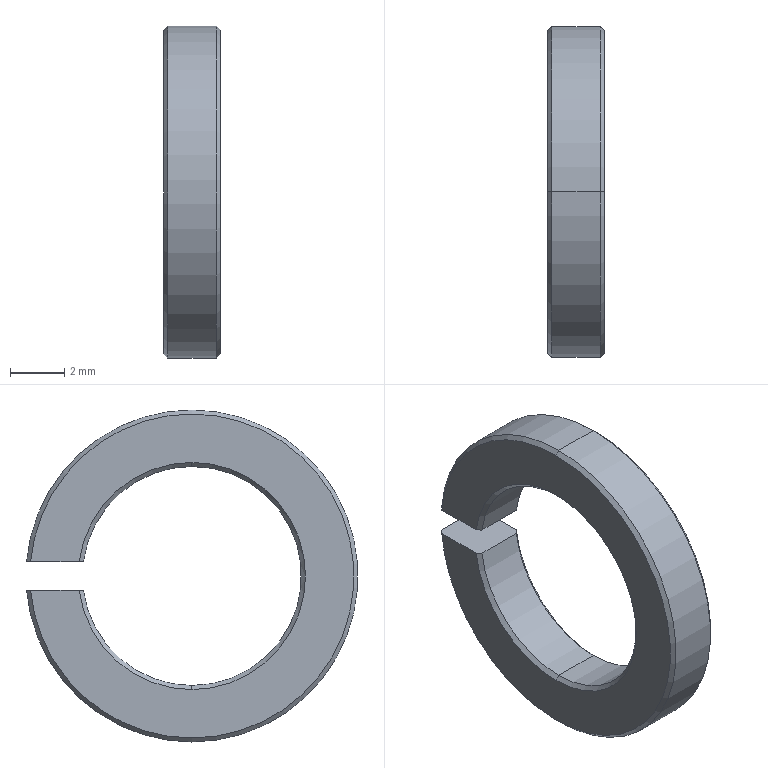Component | SolidWorks | 8_T93-1 | 1 solid | 22 faces | box 2.1 x 12.25 x 12.28 mm | volume 134 mm3 | cone 12 | cylinder 6 | plane 4 | commonest cylinder face diameters 8.1 x3 12.277 x3 | material Plain Carbon Steel
build123d program:
from build123d import *

# Parameters (mm, degrees)
EXTRUDE1_DEPTH = 2.1
CHAMFER1_SIZE  = 0.15


with BuildPart() as part:
    # Sketch1 → Extrude1 (new body)
    with BuildSketch(Plane.XY):
        with BuildLine():
            Line((-0.525, 6.116), (-0.525, 4.016))
            ThreePointArc((-0.525, 4.016), (0, -4.05), (0.525, 4.016))
            Line((0.525, 4.016), (0.525, 6.116))
            ThreePointArc((0.525, 6.116), (0, -6.138), (-0.525, 6.116))
        make_face()
    extrude(amount=EXTRUDE1_DEPTH)

    # Chamfer1
    chamfer1_edges = [part.edges().sort_by_distance(p)[0] for p in [
        (0, -4.05, 2.1),
        (0, -6.138, 2.1),
        (0, -4.05, 0),
        (0, -6.138, 0),
    ]]
    chamfer(chamfer1_edges, length=CHAMFER1_SIZE)


solid = part.part

# Placed as in the assembly
solid = solid.moved(Location((-16.1, 42.426, 42.426), (0, 90, 0)))
STEP:
#1=COLOUR_RGB('',0.7922,0.8196,0.9333);
#2=FILL_AREA_STYLE_COLOUR('',#1);
#3=FILL_AREA_STYLE('',(#2));
#4=SURFACE_STYLE_FILL_AREA(#3);
#5=SURFACE_SIDE_STYLE('',(#4));
#6=SURFACE_STYLE_USAGE(.BOTH.,#5);
#7=PRESENTATION_STYLE_ASSIGNMENT((#6));
#8=CARTESIAN_POINT('',(-0.6339,1.67,1.906));
#9=VERTEX_POINT('',#8);
#10=CARTESIAN_POINT('',(-0.6339,1.905,1.691));
#11=VERTEX_POINT('',#10);
#12=CARTESIAN_POINT('',(-0.6339,1.67,1.67));
#13=DIRECTION('',(-1.,0.,0.));
#14=DIRECTION('',(0.,0.,1.));
#15=AXIS2_PLACEMENT_3D('',#12,#13,#14);
#16=CIRCLE('',#15,0.2358);
#17=EDGE_CURVE('',#9,#11,#16,.T.);
#18=ORIENTED_EDGE('',*,*,#17,.F.);
#19=CARTESIAN_POINT('',(-0.628,1.67,1.912));
#20=VERTEX_POINT('',#19);
#21=CARTESIAN_POINT('',(-0.6339,1.67,1.906));
#22=DIRECTION('',(0.7071,0.,0.7071));
#23=VECTOR('',#22,39.37);
#24=LINE('',#21,#23);
#25=EDGE_CURVE('',#9,#20,#24,.T.);
#26=ORIENTED_EDGE('',*,*,#25,.T.);
#27=CARTESIAN_POINT('',(-0.628,1.911,1.691));
#28=VERTEX_POINT('',#27);
#29=CARTESIAN_POINT('',(-0.628,1.67,1.67));
#30=DIRECTION('',(1.,0.,0.));
#31=DIRECTION('',(0.,0.,1.));
#32=AXIS2_PLACEMENT_3D('',#29,#30,#31);
#33=CIRCLE('',#32,0.2417);
#34=EDGE_CURVE('',#28,#20,#33,.T.);
#35=ORIENTED_EDGE('',*,*,#34,.F.);
#36=CARTESIAN_POINT('',(-0.6339,1.905,1.691));
#37=CARTESIAN_POINT('',(-0.6319,1.907,1.691));
#38=CARTESIAN_POINT('',(-0.6299,1.909,1.691));
#39=CARTESIAN_POINT('',(-0.628,1.911,1.691));
#40=B_SPLINE_CURVE_WITH_KNOTS('',3,(#36,#37,#38,#39),.UNSPECIFIED.,.F.,.F.,(4,4),(0.,0.0002125),.UNSPECIFIED.);
#41=EDGE_CURVE('',#11,#28,#40,.T.);
#42=ORIENTED_EDGE('',*,*,#41,.F.);
#43=EDGE_LOOP('',(#18,#26,#35,#42));
#44=FACE_OUTER_BOUND('',#43,.T.);
#45=CARTESIAN_POINT('',(-0.6339,1.67,1.67));
#46=DIRECTION('',(1.,0.,0.));
#47=DIRECTION('',(0.,0.,-1.));
#48=AXIS2_PLACEMENT_3D('',#45,#46,#47);
#49=CONICAL_SURFACE('',#48,0.2358,0.7854);
#50=ADVANCED_FACE('',(#44),#49,.T.);
#51=ORIENTED_EDGE('',*,*,#25,.F.);
#52=CARTESIAN_POINT('',(-0.6339,1.67,1.435));
#53=VERTEX_POINT('',#52);
#54=CARTESIAN_POINT('',(-0.6339,1.67,1.67));
#55=DIRECTION('',(-1.,0.,0.));
#56=DIRECTION('',(0.,0.,1.));
#57=AXIS2_PLACEMENT_3D('',#54,#55,#56);
#58=CIRCLE('',#57,0.2358);
#59=EDGE_CURVE('',#53,#9,#58,.T.);
#60=ORIENTED_EDGE('',*,*,#59,.F.);
#61=CARTESIAN_POINT('',(-0.628,1.67,1.429));
#62=VERTEX_POINT('',#61);
#63=CARTESIAN_POINT('',(-0.6339,1.67,1.435));
#64=DIRECTION('',(0.7071,0.,-0.7071));
#65=VECTOR('',#64,39.37);
#66=LINE('',#63,#65);
#67=EDGE_CURVE('',#53,#62,#66,.T.);
#68=ORIENTED_EDGE('',*,*,#67,.T.);
#69=CARTESIAN_POINT('',(-0.628,1.67,1.67));
#70=DIRECTION('',(1.,0.,0.));
#71=DIRECTION('',(0.,0.,1.));
#72=AXIS2_PLACEMENT_3D('',#69,#70,#71);
#73=CIRCLE('',#72,0.2417);
#74=EDGE_CURVE('',#20,#62,#73,.T.);
#75=ORIENTED_EDGE('',*,*,#74,.F.);
#76=EDGE_LOOP('',(#51,#60,#68,#75));
#77=FACE_OUTER_BOUND('',#76,.T.);
#78=CARTESIAN_POINT('',(-0.6339,1.67,1.67));
#79=DIRECTION('',(1.,0.,0.));
#80=DIRECTION('',(0.,0.,-1.));
#81=AXIS2_PLACEMENT_3D('',#78,#79,#80);
#82=CONICAL_SURFACE('',#81,0.2358,0.7854);
#83=ADVANCED_FACE('',(#77),#82,.T.);
#84=CARTESIAN_POINT('',(-0.628,1.67,1.511));
#85=VERTEX_POINT('',#84);
#86=CARTESIAN_POINT('',(-0.628,1.67,1.83));
#87=VERTEX_POINT('',#86);
#88=CARTESIAN_POINT('',(-0.628,1.67,1.67));
#89=DIRECTION('',(-1.,0.,0.));
#90=DIRECTION('',(0.,0.,1.));
#91=AXIS2_PLACEMENT_3D('',#88,#89,#90);
#92=CIRCLE('',#91,0.1594);
#93=EDGE_CURVE('',#85,#87,#92,.T.);
#94=ORIENTED_EDGE('',*,*,#93,.F.);
#95=CARTESIAN_POINT('',(-0.6339,1.67,1.505));
#96=VERTEX_POINT('',#95);
#97=CARTESIAN_POINT('',(-0.6339,1.67,1.505));
#98=DIRECTION('',(-0.7071,0.,-0.7071));
#99=VECTOR('',#98,39.37);
#100=LINE('',#97,#99);
#101=EDGE_CURVE('',#85,#96,#100,.T.);
#102=ORIENTED_EDGE('',*,*,#101,.T.);
#103=CARTESIAN_POINT('',(-0.6339,1.67,1.836));
#104=VERTEX_POINT('',#103);
#105=CARTESIAN_POINT('',(-0.6339,1.67,1.67));
#106=DIRECTION('',(1.,0.,0.));
#107=DIRECTION('',(0.,0.,1.));
#108=AXIS2_PLACEMENT_3D('',#105,#106,#107);
#109=CIRCLE('',#108,0.1654);
#110=EDGE_CURVE('',#104,#96,#109,.T.);
#111=ORIENTED_EDGE('',*,*,#110,.F.);
#112=CARTESIAN_POINT('',(-0.6339,1.67,1.836));
#113=DIRECTION('',(-0.7071,0.,0.7071));
#114=VECTOR('',#113,39.37);
#115=LINE('',#112,#114);
#116=EDGE_CURVE('',#87,#104,#115,.T.);
#117=ORIENTED_EDGE('',*,*,#116,.F.);
#118=EDGE_LOOP('',(#94,#102,#111,#117));
#119=FACE_OUTER_BOUND('',#118,.T.);
#120=CARTESIAN_POINT('',(-0.6339,1.67,1.67));
#121=DIRECTION('',(-1.,0.,0.));
#122=DIRECTION('',(0.,0.,1.));
#123=AXIS2_PLACEMENT_3D('',#120,#121,#122);
#124=CONICAL_SURFACE('',#123,0.1654,0.7854);
#125=ADVANCED_FACE('',(#119),#124,.F.);
#126=CARTESIAN_POINT('',(-0.628,1.828,1.691));
#127=VERTEX_POINT('',#126);
#128=CARTESIAN_POINT('',(-0.628,1.67,1.67));
#129=DIRECTION('',(-1.,0.,0.));
#130=DIRECTION('',(0.,0.,1.));
#131=AXIS2_PLACEMENT_3D('',#128,#129,#130);
#132=CIRCLE('',#131,0.1594);
#133=EDGE_CURVE('',#87,#127,#132,.T.);
#134=ORIENTED_EDGE('',*,*,#133,.F.);
#135=ORIENTED_EDGE('',*,*,#116,.T.);
#136=CARTESIAN_POINT('',(-0.6339,1.834,1.691));
#137=VERTEX_POINT('',#136);
#138=CARTESIAN_POINT('',(-0.6339,1.67,1.67));
#139=DIRECTION('',(1.,0.,0.));
#140=DIRECTION('',(0.,-0.,1.));
#141=AXIS2_PLACEMENT_3D('',#138,#139,#140);
#142=CIRCLE('',#141,0.1654);
#143=EDGE_CURVE('',#137,#104,#142,.T.);
#144=ORIENTED_EDGE('',*,*,#143,.F.);
#145=CARTESIAN_POINT('',(-0.628,1.828,1.691));
#146=CARTESIAN_POINT('',(-0.6299,1.83,1.691));
#147=CARTESIAN_POINT('',(-0.6319,1.832,1.691));
#148=CARTESIAN_POINT('',(-0.6339,1.834,1.691));
#149=B_SPLINE_CURVE_WITH_KNOTS('',3,(#145,#146,#147,#148),.UNSPECIFIED.,.F.,.F.,(4,4),(0.,0.000213),.UNSPECIFIED.);
#150=EDGE_CURVE('',#127,#137,#149,.T.);
#151=ORIENTED_EDGE('',*,*,#150,.F.);
#152=EDGE_LOOP('',(#134,#135,#144,#151));
#153=FACE_OUTER_BOUND('',#152,.T.);
#154=CARTESIAN_POINT('',(-0.6339,1.67,1.67));
#155=DIRECTION('',(-1.,0.,0.));
#156=DIRECTION('',(0.,0.,1.));
#157=AXIS2_PLACEMENT_3D('',#154,#155,#156);
#158=CONICAL_SURFACE('',#157,0.1654,0.7854);
#159=ADVANCED_FACE('',(#153),#158,.F.);
#160=CARTESIAN_POINT('',(-0.5571,1.67,1.83));
#161=VERTEX_POINT('',#160);
#162=CARTESIAN_POINT('',(-0.5571,1.67,1.511));
#163=VERTEX_POINT('',#162);
#164=CARTESIAN_POINT('',(-0.5571,1.67,1.67));
#165=DIRECTION('',(1.,0.,0.));
#166=DIRECTION('',(0.,0.,1.));
#167=AXIS2_PLACEMENT_3D('',#164,#165,#166);
#168=CIRCLE('',#167,0.1594);
#169=EDGE_CURVE('',#161,#163,#168,.T.);
#170=ORIENTED_EDGE('',*,*,#169,.F.);
#171=CARTESIAN_POINT('',(-0.5512,1.67,1.836));
#172=VERTEX_POINT('',#171);
#173=CARTESIAN_POINT('',(-0.5571,1.67,1.83));
#174=DIRECTION('',(0.7071,0.,0.7071));
#175=VECTOR('',#174,39.37);
#176=LINE('',#173,#175);
#177=EDGE_CURVE('',#161,#172,#176,.T.);
#178=ORIENTED_EDGE('',*,*,#177,.T.);
#179=CARTESIAN_POINT('',(-0.5512,1.67,1.505));
#180=VERTEX_POINT('',#179);
#181=CARTESIAN_POINT('',(-0.5512,1.67,1.67));
#182=DIRECTION('',(-1.,0.,0.));
#183=DIRECTION('',(0.,0.,1.));
#184=AXIS2_PLACEMENT_3D('',#181,#182,#183);
#185=CIRCLE('',#184,0.1654);
#186=EDGE_CURVE('',#180,#172,#185,.T.);
#187=ORIENTED_EDGE('',*,*,#186,.F.);
#188=CARTESIAN_POINT('',(-0.5571,1.67,1.511));
#189=DIRECTION('',(0.7071,0.,-0.7071));
#190=VECTOR('',#189,39.37);
#191=LINE('',#188,#190);
#192=EDGE_CURVE('',#163,#180,#191,.T.);
#193=ORIENTED_EDGE('',*,*,#192,.F.);
#194=EDGE_LOOP('',(#170,#178,#187,#193));
#195=FACE_OUTER_BOUND('',#194,.T.);
#196=CARTESIAN_POINT('',(-0.5571,1.67,1.67));
#197=DIRECTION('',(1.,0.,0.));
#198=DIRECTION('',(0.,0.,-1.));
#199=AXIS2_PLACEMENT_3D('',#196,#197,#198);
#200=CONICAL_SURFACE('',#199,0.1594,0.7854);
#201=ADVANCED_FACE('',(#195),#200,.F.);
#202=CARTESIAN_POINT('',(-0.5571,1.828,1.65));
#203=VERTEX_POINT('',#202);
#204=CARTESIAN_POINT('',(-0.5571,1.67,1.67));
#205=DIRECTION('',(1.,0.,0.));
#206=DIRECTION('',(0.,0.,1.));
#207=AXIS2_PLACEMENT_3D('',#204,#205,#206);
#208=CIRCLE('',#207,0.1594);
#209=EDGE_CURVE('',#163,#203,#208,.T.);
#210=ORIENTED_EDGE('',*,*,#209,.F.);
#211=ORIENTED_EDGE('',*,*,#192,.T.);
#212=CARTESIAN_POINT('',(-0.5512,1.834,1.65));
#213=VERTEX_POINT('',#212);
#214=CARTESIAN_POINT('',(-0.5512,1.67,1.67));
#215=DIRECTION('',(-1.,0.,0.));
#216=DIRECTION('',(0.,0.,1.));
#217=AXIS2_PLACEMENT_3D('',#214,#215,#216);
#218=CIRCLE('',#217,0.1654);
#219=EDGE_CURVE('',#213,#180,#218,.T.);
#220=ORIENTED_EDGE('',*,*,#219,.F.);
#221=CARTESIAN_POINT('',(-0.5571,1.828,1.65));
#222=CARTESIAN_POINT('',(-0.5551,1.83,1.65));
#223=CARTESIAN_POINT('',(-0.5531,1.832,1.65));
#224=CARTESIAN_POINT('',(-0.5512,1.834,1.65));
#225=B_SPLINE_CURVE_WITH_KNOTS('',3,(#221,#222,#223,#224),.UNSPECIFIED.,.F.,.F.,(4,4),(0.,0.000213),.UNSPECIFIED.);
#226=EDGE_CURVE('',#203,#213,#225,.T.);
#227=ORIENTED_EDGE('',*,*,#226,.F.);
#228=EDGE_LOOP('',(#210,#211,#220,#227));
#229=FACE_OUTER_BOUND('',#228,.T.);
#230=CARTESIAN_POINT('',(-0.5571,1.67,1.67));
#231=DIRECTION('',(1.,0.,0.));
#232=DIRECTION('',(0.,0.,-1.));
#233=AXIS2_PLACEMENT_3D('',#230,#231,#232);
#234=CONICAL_SURFACE('',#233,0.1594,0.7854);
#235=ADVANCED_FACE('',(#229),#234,.F.);
#236=CARTESIAN_POINT('',(-0.5512,1.67,1.435));
#237=VERTEX_POINT('',#236);
#238=CARTESIAN_POINT('',(-0.5512,1.905,1.65));
#239=VERTEX_POINT('',#238);
#240=CARTESIAN_POINT('',(-0.5512,1.67,1.67));
#241=DIRECTION('',(1.,0.,0.));
#242=DIRECTION('',(0.,0.,1.));
#243=AXIS2_PLACEMENT_3D('',#240,#241,#242);
#244=CIRCLE('',#243,0.2358);
#245=EDGE_CURVE('',#237,#239,#244,.T.);
#246=ORIENTED_EDGE('',*,*,#245,.F.);
#247=CARTESIAN_POINT('',(-0.5571,1.67,1.429));
#248=VERTEX_POINT('',#247);
#249=CARTESIAN_POINT('',(-0.5571,1.67,1.429));
#250=DIRECTION('',(-0.7071,0.,-0.7071));
#251=VECTOR('',#250,39.37);
#252=LINE('',#249,#251);
#253=EDGE_CURVE('',#237,#248,#252,.T.);
#254=ORIENTED_EDGE('',*,*,#253,.T.);
#255=CARTESIAN_POINT('',(-0.5571,1.911,1.65));
#256=VERTEX_POINT('',#255);
#257=CARTESIAN_POINT('',(-0.5571,1.67,1.67));
#258=DIRECTION('',(-1.,0.,0.));
#259=DIRECTION('',(0.,0.,1.));
#260=AXIS2_PLACEMENT_3D('',#257,#258,#259);
#261=CIRCLE('',#260,0.2417);
#262=EDGE_CURVE('',#256,#248,#261,.T.);
#263=ORIENTED_EDGE('',*,*,#262,.F.);
#264=CARTESIAN_POINT('',(-0.5512,1.905,1.65));
#265=CARTESIAN_POINT('',(-0.5531,1.907,1.65));
#266=CARTESIAN_POINT('',(-0.5551,1.909,1.65));
#267=CARTESIAN_POINT('',(-0.5571,1.911,1.65));
#268=B_SPLINE_CURVE_WITH_KNOTS('',3,(#264,#265,#266,#267),.UNSPECIFIED.,.F.,.F.,(4,4),(0.,0.0002125),.UNSPECIFIED.);
#269=EDGE_CURVE('',#239,#256,#268,.T.);
#270=ORIENTED_EDGE('',*,*,#269,.F.);
#271=EDGE_LOOP('',(#246,#254,#263,#270));
#272=FACE_OUTER_BOUND('',#271,.T.);
#273=CARTESIAN_POINT('',(-0.5571,1.67,1.67));
#274=DIRECTION('',(-1.,0.,0.));
#275=DIRECTION('',(0.,0.,1.));
#276=AXIS2_PLACEMENT_3D('',#273,#274,#275);
#277=CONICAL_SURFACE('',#276,0.2417,0.7854);
#278=ADVANCED_FACE('',(#272),#277,.T.);
#279=ORIENTED_EDGE('',*,*,#253,.F.);
#280=CARTESIAN_POINT('',(-0.5512,1.67,1.906));
#281=VERTEX_POINT('',#280);
#282=CARTESIAN_POINT('',(-0.5512,1.67,1.67));
#283=DIRECTION('',(1.,0.,0.));
#284=DIRECTION('',(0.,0.,1.));
#285=AXIS2_PLACEMENT_3D('',#282,#283,#284);
#286=CIRCLE('',#285,0.2358);
#287=EDGE_CURVE('',#281,#237,#286,.T.);
#288=ORIENTED_EDGE('',*,*,#287,.F.);
#289=CARTESIAN_POINT('',(-0.5571,1.67,1.912));
#290=VERTEX_POINT('',#289);
#291=CARTESIAN_POINT('',(-0.5571,1.67,1.912));
#292=DIRECTION('',(-0.7071,0.,0.7071));
#293=VECTOR('',#292,39.37);
#294=LINE('',#291,#293);
#295=EDGE_CURVE('',#281,#290,#294,.T.);
#296=ORIENTED_EDGE('',*,*,#295,.T.);
#297=CARTESIAN_POINT('',(-0.5571,1.67,1.67));
#298=DIRECTION('',(-1.,0.,0.));
#299=DIRECTION('',(0.,0.,1.));
#300=AXIS2_PLACEMENT_3D('',#297,#298,#299);
#301=CIRCLE('',#300,0.2417);
#302=EDGE_CURVE('',#248,#290,#301,.T.);
#303=ORIENTED_EDGE('',*,*,#302,.F.);
#304=EDGE_LOOP('',(#279,#288,#296,#303));
#305=FACE_OUTER_BOUND('',#304,.T.);
#306=CARTESIAN_POINT('',(-0.5571,1.67,1.67));
#307=DIRECTION('',(-1.,0.,0.));
#308=DIRECTION('',(0.,0.,1.));
#309=AXIS2_PLACEMENT_3D('',#306,#307,#308);
#310=CONICAL_SURFACE('',#309,0.2417,0.7854);
#311=ADVANCED_FACE('',(#305),#310,.T.);
#312=ORIENTED_EDGE('',*,*,#93,.T.);
#313=CARTESIAN_POINT('',(-0.6339,1.67,1.83));
#314=DIRECTION('',(1.,0.,0.));
#315=VECTOR('',#314,39.37);
#316=LINE('',#313,#315);
#317=EDGE_CURVE('',#87,#161,#316,.T.);
#318=ORIENTED_EDGE('',*,*,#317,.T.);
#319=ORIENTED_EDGE('',*,*,#169,.T.);
#320=CARTESIAN_POINT('',(-0.6339,1.67,1.511));
#321=DIRECTION('',(1.,0.,0.));
#322=VECTOR('',#321,39.37);
#323=LINE('',#320,#322);
#324=EDGE_CURVE('',#85,#163,#323,.T.);
#325=ORIENTED_EDGE('',*,*,#324,.F.);
#326=EDGE_LOOP('',(#312,#318,#319,#325));
#327=FACE_OUTER_BOUND('',#326,.T.);
#328=CARTESIAN_POINT('',(-0.6339,1.67,1.67));
#329=DIRECTION('',(1.,0.,0.));
#330=DIRECTION('',(0.,0.,-1.));
#331=AXIS2_PLACEMENT_3D('',#328,#329,#330);
#332=CYLINDRICAL_SURFACE('',#331,0.1594);
#333=ADVANCED_FACE('',(#327),#332,.F.);
#334=CARTESIAN_POINT('',(-0.628,1.828,1.65));
#335=VERTEX_POINT('',#334);
#336=CARTESIAN_POINT('',(-0.628,1.67,1.67));
#337=DIRECTION('',(-1.,0.,0.));
#338=DIRECTION('',(0.,0.,1.));
#339=AXIS2_PLACEMENT_3D('',#336,#337,#338);
#340=CIRCLE('',#339,0.1594);
#341=EDGE_CURVE('',#335,#85,#340,.T.);
#342=ORIENTED_EDGE('',*,*,#341,.T.);
#343=ORIENTED_EDGE('',*,*,#324,.T.);
#344=ORIENTED_EDGE('',*,*,#209,.T.);
#345=CARTESIAN_POINT('',(-0.6339,1.828,1.65));
#346=DIRECTION('',(1.,0.,0.));
#347=VECTOR('',#346,39.37);
#348=LINE('',#345,#347);
#349=EDGE_CURVE('',#335,#203,#348,.T.);
#350=ORIENTED_EDGE('',*,*,#349,.F.);
#351=EDGE_LOOP('',(#342,#343,#344,#350));
#352=FACE_OUTER_BOUND('',#351,.T.);
#353=CARTESIAN_POINT('',(-0.6339,1.67,1.67));
#354=DIRECTION('',(1.,0.,0.));
#355=DIRECTION('',(0.,0.,-1.));
#356=AXIS2_PLACEMENT_3D('',#353,#354,#355);
#357=CYLINDRICAL_SURFACE('',#356,0.1594);
#358=ADVANCED_FACE('',(#352),#357,.F.);
#359=ORIENTED_EDGE('',*,*,#34,.T.);
#360=CARTESIAN_POINT('',(-0.6339,1.67,1.912));
#361=DIRECTION('',(1.,0.,0.));
#362=VECTOR('',#361,39.37);
#363=LINE('',#360,#362);
#364=EDGE_CURVE('',#20,#290,#363,.T.);
#365=ORIENTED_EDGE('',*,*,#364,.T.);
#366=CARTESIAN_POINT('',(-0.5571,1.911,1.691));
#367=VERTEX_POINT('',#366);
#368=CARTESIAN_POINT('',(-0.5571,1.67,1.67));
#369=DIRECTION('',(-1.,0.,0.));
#370=DIRECTION('',(0.,0.,1.));
#371=AXIS2_PLACEMENT_3D('',#368,#369,#370);
#372=CIRCLE('',#371,0.2417);
#373=EDGE_CURVE('',#290,#367,#372,.T.);
#374=ORIENTED_EDGE('',*,*,#373,.T.);
#375=CARTESIAN_POINT('',(-0.6339,1.911,1.691));
#376=DIRECTION('',(1.,0.,0.));
#377=VECTOR('',#376,39.37);
#378=LINE('',#375,#377);
#379=EDGE_CURVE('',#28,#367,#378,.T.);
#380=ORIENTED_EDGE('',*,*,#379,.F.);
#381=EDGE_LOOP('',(#359,#365,#374,#380));
#382=FACE_OUTER_BOUND('',#381,.T.);
#383=CARTESIAN_POINT('',(-0.6339,1.67,1.67));
#384=DIRECTION('',(1.,0.,0.));
#385=DIRECTION('',(0.,0.,-1.));
#386=AXIS2_PLACEMENT_3D('',#383,#384,#385);
#387=CYLINDRICAL_SURFACE('',#386,0.2417);
#388=ADVANCED_FACE('',(#382),#387,.T.);
#389=ORIENTED_EDGE('',*,*,#364,.F.);
#390=ORIENTED_EDGE('',*,*,#74,.T.);
#391=CARTESIAN_POINT('',(-0.6339,1.67,1.429));
#392=DIRECTION('',(1.,0.,0.));
#393=VECTOR('',#392,39.37);
#394=LINE('',#391,#393);
#395=EDGE_CURVE('',#62,#248,#394,.T.);
#396=ORIENTED_EDGE('',*,*,#395,.T.);
#397=ORIENTED_EDGE('',*,*,#302,.T.);
#398=EDGE_LOOP('',(#389,#390,#396,#397));
#399=FACE_OUTER_BOUND('',#398,.T.);
#400=CARTESIAN_POINT('',(-0.6339,1.67,1.67));
#401=DIRECTION('',(1.,0.,0.));
#402=DIRECTION('',(0.,0.,-1.));
#403=AXIS2_PLACEMENT_3D('',#400,#401,#402);
#404=CYLINDRICAL_SURFACE('',#403,0.2417);
#405=ADVANCED_FACE('',(#399),#404,.T.);
#406=ORIENTED_EDGE('',*,*,#395,.F.);
#407=CARTESIAN_POINT('',(-0.628,1.911,1.65));
#408=VERTEX_POINT('',#407);
#409=CARTESIAN_POINT('',(-0.628,1.67,1.67));
#410=DIRECTION('',(1.,0.,0.));
#411=DIRECTION('',(0.,0.,1.));
#412=AXIS2_PLACEMENT_3D('',#409,#410,#411);
#413=CIRCLE('',#412,0.2417);
#414=EDGE_CURVE('',#62,#408,#413,.T.);
#415=ORIENTED_EDGE('',*,*,#414,.T.);
#416=CARTESIAN_POINT('',(-0.6339,1.911,1.65));
#417=DIRECTION('',(1.,0.,0.));
#418=VECTOR('',#417,39.37);
#419=LINE('',#416,#418);
#420=EDGE_CURVE('',#408,#256,#419,.T.);
#421=ORIENTED_EDGE('',*,*,#420,.T.);
#422=ORIENTED_EDGE('',*,*,#262,.T.);
#423=EDGE_LOOP('',(#406,#415,#421,#422));
#424=FACE_OUTER_BOUND('',#423,.T.);
#425=CARTESIAN_POINT('',(-0.6339,1.67,1.67));
#426=DIRECTION('',(1.,0.,0.));
#427=DIRECTION('',(0.,0.,-1.));
#428=AXIS2_PLACEMENT_3D('',#425,#426,#427);
#429=CYLINDRICAL_SURFACE('',#428,0.2417);
#430=ADVANCED_FACE('',(#424),#429,.T.);
#431=ORIENTED_EDGE('',*,*,#379,.T.);
#432=CARTESIAN_POINT('',(-0.5512,1.905,1.691));
#433=VERTEX_POINT('',#432);
#434=CARTESIAN_POINT('',(-0.5571,1.911,1.691));
#435=CARTESIAN_POINT('',(-0.5551,1.909,1.691));
#436=CARTESIAN_POINT('',(-0.5531,1.907,1.691));
#437=CARTESIAN_POINT('',(-0.5512,1.905,1.691));
#438=B_SPLINE_CURVE_WITH_KNOTS('',3,(#434,#435,#436,#437),.UNSPECIFIED.,.F.,.F.,(4,4),(0.,0.0002125),.UNSPECIFIED.);
#439=EDGE_CURVE('',#367,#433,#438,.T.);
#440=ORIENTED_EDGE('',*,*,#439,.T.);
#441=CARTESIAN_POINT('',(-0.5512,1.834,1.691));
#442=VERTEX_POINT('',#441);
#443=CARTESIAN_POINT('',(-0.5512,1.911,1.691));
#444=DIRECTION('',(0.,-1.,0.));
#445=VECTOR('',#444,39.37);
#446=LINE('',#443,#445);
#447=EDGE_CURVE('',#433,#442,#446,.T.);
#448=ORIENTED_EDGE('',*,*,#447,.T.);
#449=CARTESIAN_POINT('',(-0.5571,1.828,1.691));
#450=VERTEX_POINT('',#449);
#451=CARTESIAN_POINT('',(-0.5512,1.834,1.691));
#452=CARTESIAN_POINT('',(-0.5531,1.832,1.691));
#453=CARTESIAN_POINT('',(-0.5551,1.83,1.691));
#454=CARTESIAN_POINT('',(-0.5571,1.828,1.691));
#455=B_SPLINE_CURVE_WITH_KNOTS('',3,(#451,#452,#453,#454),.UNSPECIFIED.,.F.,.F.,(4,4),(0.,0.000213),.UNSPECIFIED.);
#456=EDGE_CURVE('',#442,#450,#455,.T.);
#457=ORIENTED_EDGE('',*,*,#456,.T.);
#458=CARTESIAN_POINT('',(-0.6339,1.828,1.691));
#459=DIRECTION('',(1.,0.,0.));
#460=VECTOR('',#459,39.37);
#461=LINE('',#458,#460);
#462=EDGE_CURVE('',#127,#450,#461,.T.);
#463=ORIENTED_EDGE('',*,*,#462,.F.);
#464=ORIENTED_EDGE('',*,*,#150,.T.);
#465=CARTESIAN_POINT('',(-0.6339,1.911,1.691));
#466=DIRECTION('',(0.,-1.,0.));
#467=VECTOR('',#466,39.37);
#468=LINE('',#465,#467);
#469=EDGE_CURVE('',#11,#137,#468,.T.);
#470=ORIENTED_EDGE('',*,*,#469,.F.);
#471=ORIENTED_EDGE('',*,*,#41,.T.);
#472=EDGE_LOOP('',(#431,#440,#448,#457,#463,#464,#470,#471));
#473=FACE_OUTER_BOUND('',#472,.T.);
#474=CARTESIAN_POINT('',(-0.6339,1.911,1.691));
#475=DIRECTION('',(0.,0.,1.));
#476=DIRECTION('',(0.,1.,-0.));
#477=AXIS2_PLACEMENT_3D('',#474,#475,#476);
#478=PLANE('',#477);
#479=ADVANCED_FACE('',(#473),#478,.F.);
#480=ORIENTED_EDGE('',*,*,#317,.F.);
#481=ORIENTED_EDGE('',*,*,#133,.T.);
#482=ORIENTED_EDGE('',*,*,#462,.T.);
#483=CARTESIAN_POINT('',(-0.5571,1.67,1.67));
#484=DIRECTION('',(1.,0.,0.));
#485=DIRECTION('',(0.,0.,1.));
#486=AXIS2_PLACEMENT_3D('',#483,#484,#485);
#487=CIRCLE('',#486,0.1594);
#488=EDGE_CURVE('',#450,#161,#487,.T.);
#489=ORIENTED_EDGE('',*,*,#488,.T.);
#490=EDGE_LOOP('',(#480,#481,#482,#489));
#491=FACE_OUTER_BOUND('',#490,.T.);
#492=CARTESIAN_POINT('',(-0.6339,1.67,1.67));
#493=DIRECTION('',(1.,0.,0.));
#494=DIRECTION('',(0.,0.,-1.));
#495=AXIS2_PLACEMENT_3D('',#492,#493,#494);
#496=CYLINDRICAL_SURFACE('',#495,0.1594);
#497=ADVANCED_FACE('',(#491),#496,.F.);
#498=CARTESIAN_POINT('',(-0.5512,1.911,1.65));
#499=DIRECTION('',(0.,1.,-0.));
#500=VECTOR('',#499,39.37);
#501=LINE('',#498,#500);
#502=EDGE_CURVE('',#213,#239,#501,.T.);
#503=ORIENTED_EDGE('',*,*,#502,.T.);
#504=ORIENTED_EDGE('',*,*,#269,.T.);
#505=ORIENTED_EDGE('',*,*,#420,.F.);
#506=CARTESIAN_POINT('',(-0.6339,1.905,1.65));
#507=VERTEX_POINT('',#506);
#508=CARTESIAN_POINT('',(-0.628,1.911,1.65));
#509=CARTESIAN_POINT('',(-0.6299,1.909,1.65));
#510=CARTESIAN_POINT('',(-0.6319,1.907,1.65));
#511=CARTESIAN_POINT('',(-0.6339,1.905,1.65));
#512=B_SPLINE_CURVE_WITH_KNOTS('',3,(#508,#509,#510,#511),.UNSPECIFIED.,.F.,.F.,(4,4),(0.,0.0002125),.UNSPECIFIED.);
#513=EDGE_CURVE('',#408,#507,#512,.T.);
#514=ORIENTED_EDGE('',*,*,#513,.T.);
#515=CARTESIAN_POINT('',(-0.6339,1.834,1.65));
#516=VERTEX_POINT('',#515);
#517=CARTESIAN_POINT('',(-0.6339,1.911,1.65));
#518=DIRECTION('',(0.,1.,-0.));
#519=VECTOR('',#518,39.37);
#520=LINE('',#517,#519);
#521=EDGE_CURVE('',#516,#507,#520,.T.);
#522=ORIENTED_EDGE('',*,*,#521,.F.);
#523=CARTESIAN_POINT('',(-0.6339,1.834,1.65));
#524=CARTESIAN_POINT('',(-0.6319,1.832,1.65));
#525=CARTESIAN_POINT('',(-0.6299,1.83,1.65));
#526=CARTESIAN_POINT('',(-0.628,1.828,1.65));
#527=B_SPLINE_CURVE_WITH_KNOTS('',3,(#523,#524,#525,#526),.UNSPECIFIED.,.F.,.F.,(4,4),(0.,0.000213),.UNSPECIFIED.);
#528=EDGE_CURVE('',#516,#335,#527,.T.);
#529=ORIENTED_EDGE('',*,*,#528,.T.);
#530=ORIENTED_EDGE('',*,*,#349,.T.);
#531=ORIENTED_EDGE('',*,*,#226,.T.);
#532=EDGE_LOOP('',(#503,#504,#505,#514,#522,#529,#530,#531));
#533=FACE_OUTER_BOUND('',#532,.T.);
#534=CARTESIAN_POINT('',(-0.6339,1.911,1.65));
#535=DIRECTION('',(0.,-0.,-1.));
#536=DIRECTION('',(0.,-1.,0.));
#537=AXIS2_PLACEMENT_3D('',#534,#535,#536);
#538=PLANE('',#537);
#539=ADVANCED_FACE('',(#533),#538,.F.);
#540=ORIENTED_EDGE('',*,*,#469,.T.);
#541=ORIENTED_EDGE('',*,*,#143,.T.);
#542=ORIENTED_EDGE('',*,*,#110,.T.);
#543=CARTESIAN_POINT('',(-0.6339,1.67,1.67));
#544=DIRECTION('',(1.,0.,0.));
#545=DIRECTION('',(0.,0.,1.));
#546=AXIS2_PLACEMENT_3D('',#543,#544,#545);
#547=CIRCLE('',#546,0.1654);
#548=EDGE_CURVE('',#96,#516,#547,.T.);
#549=ORIENTED_EDGE('',*,*,#548,.T.);
#550=ORIENTED_EDGE('',*,*,#521,.T.);
#551=CARTESIAN_POINT('',(-0.6339,1.67,1.67));
#552=DIRECTION('',(-1.,0.,0.));
#553=DIRECTION('',(0.,0.,1.));
#554=AXIS2_PLACEMENT_3D('',#551,#552,#553);
#555=CIRCLE('',#554,0.2358);
#556=EDGE_CURVE('',#507,#53,#555,.T.);
#557=ORIENTED_EDGE('',*,*,#556,.T.);
#558=ORIENTED_EDGE('',*,*,#59,.T.);
#559=ORIENTED_EDGE('',*,*,#17,.T.);
#560=EDGE_LOOP('',(#540,#541,#542,#549,#550,#557,#558,#559));
#561=FACE_OUTER_BOUND('',#560,.T.);
#562=CARTESIAN_POINT('',(-0.6339,1.67,1.67));
#563=DIRECTION('',(-1.,0.,0.));
#564=DIRECTION('',(0.,0.,1.));
#565=AXIS2_PLACEMENT_3D('',#562,#563,#564);
#566=PLANE('',#565);
#567=ADVANCED_FACE('',(#561),#566,.T.);
#568=ORIENTED_EDGE('',*,*,#447,.F.);
#569=CARTESIAN_POINT('',(-0.5512,1.67,1.67));
#570=DIRECTION('',(1.,0.,0.));
#571=DIRECTION('',(0.,0.,1.));
#572=AXIS2_PLACEMENT_3D('',#569,#570,#571);
#573=CIRCLE('',#572,0.2358);
#574=EDGE_CURVE('',#433,#281,#573,.T.);
#575=ORIENTED_EDGE('',*,*,#574,.T.);
#576=ORIENTED_EDGE('',*,*,#287,.T.);
#577=ORIENTED_EDGE('',*,*,#245,.T.);
#578=ORIENTED_EDGE('',*,*,#502,.F.);
#579=ORIENTED_EDGE('',*,*,#219,.T.);
#580=ORIENTED_EDGE('',*,*,#186,.T.);
#581=CARTESIAN_POINT('',(-0.5512,1.67,1.67));
#582=DIRECTION('',(-1.,0.,0.));
#583=DIRECTION('',(0.,0.,1.));
#584=AXIS2_PLACEMENT_3D('',#581,#582,#583);
#585=CIRCLE('',#584,0.1654);
#586=EDGE_CURVE('',#172,#442,#585,.T.);
#587=ORIENTED_EDGE('',*,*,#586,.T.);
#588=EDGE_LOOP('',(#568,#575,#576,#577,#578,#579,#580,#587));
#589=FACE_OUTER_BOUND('',#588,.T.);
#590=CARTESIAN_POINT('',(-0.5512,1.67,1.67));
#591=DIRECTION('',(-1.,0.,0.));
#592=DIRECTION('',(0.,0.,1.));
#593=AXIS2_PLACEMENT_3D('',#590,#591,#592);
#594=PLANE('',#593);
#595=ADVANCED_FACE('',(#589),#594,.F.);
#596=ORIENTED_EDGE('',*,*,#295,.F.);
#597=ORIENTED_EDGE('',*,*,#574,.F.);
#598=ORIENTED_EDGE('',*,*,#439,.F.);
#599=ORIENTED_EDGE('',*,*,#373,.F.);
#600=EDGE_LOOP('',(#596,#597,#598,#599));
#601=FACE_OUTER_BOUND('',#600,.T.);
#602=CARTESIAN_POINT('',(-0.5571,1.67,1.67));
#603=DIRECTION('',(-1.,0.,0.));
#604=DIRECTION('',(0.,0.,1.));
#605=AXIS2_PLACEMENT_3D('',#602,#603,#604);
#606=CONICAL_SURFACE('',#605,0.2417,0.7854);
#607=ADVANCED_FACE('',(#601),#606,.T.);
#608=ORIENTED_EDGE('',*,*,#177,.F.);
#609=ORIENTED_EDGE('',*,*,#488,.F.);
#610=ORIENTED_EDGE('',*,*,#456,.F.);
#611=ORIENTED_EDGE('',*,*,#586,.F.);
#612=EDGE_LOOP('',(#608,#609,#610,#611));
#613=FACE_OUTER_BOUND('',#612,.T.);
#614=CARTESIAN_POINT('',(-0.5571,1.67,1.67));
#615=DIRECTION('',(1.,0.,0.));
#616=DIRECTION('',(0.,0.,-1.));
#617=AXIS2_PLACEMENT_3D('',#614,#615,#616);
#618=CONICAL_SURFACE('',#617,0.1594,0.7854);
#619=ADVANCED_FACE('',(#613),#618,.F.);
#620=ORIENTED_EDGE('',*,*,#101,.F.);
#621=ORIENTED_EDGE('',*,*,#341,.F.);
#622=ORIENTED_EDGE('',*,*,#528,.F.);
#623=ORIENTED_EDGE('',*,*,#548,.F.);
#624=EDGE_LOOP('',(#620,#621,#622,#623));
#625=FACE_OUTER_BOUND('',#624,.T.);
#626=CARTESIAN_POINT('',(-0.6339,1.67,1.67));
#627=DIRECTION('',(-1.,0.,0.));
#628=DIRECTION('',(0.,0.,1.));
#629=AXIS2_PLACEMENT_3D('',#626,#627,#628);
#630=CONICAL_SURFACE('',#629,0.1654,0.7854);
#631=ADVANCED_FACE('',(#625),#630,.F.);
#632=ORIENTED_EDGE('',*,*,#67,.F.);
#633=ORIENTED_EDGE('',*,*,#556,.F.);
#634=ORIENTED_EDGE('',*,*,#513,.F.);
#635=ORIENTED_EDGE('',*,*,#414,.F.);
#636=EDGE_LOOP('',(#632,#633,#634,#635));
#637=FACE_OUTER_BOUND('',#636,.T.);
#638=CARTESIAN_POINT('',(-0.6339,1.67,1.67));
#639=DIRECTION('',(1.,0.,0.));
#640=DIRECTION('',(0.,0.,-1.));
#641=AXIS2_PLACEMENT_3D('',#638,#639,#640);
#642=CONICAL_SURFACE('',#641,0.2358,0.7854);
#643=ADVANCED_FACE('',(#637),#642,.T.);
#644=CLOSED_SHELL('',(#50,#83,#125,#159,#201,#235,#278,#311,#333,#358,#388,#405,#430,#479,#497,#539,#567,#595,#607,#619,#631,#643));
#645=MANIFOLD_SOLID_BREP('',#644);
#646=STYLED_ITEM('',(#7),#645);
#647=PRESENTATION_LAYER_ASSIGNMENT('','',(#646));
#648=(LENGTH_UNIT()NAMED_UNIT(*)SI_UNIT($,.METRE.));
#649=LENGTH_MEASURE_WITH_UNIT(LENGTH_MEASURE(0.0254),#648);
#650=DIMENSIONAL_EXPONENTS(1.,0.,0.,0.,0.,0.,0.);
#651=(CONVERSION_BASED_UNIT('',#649)LENGTH_UNIT()NAMED_UNIT(#650));
#652=UNCERTAINTY_MEASURE_WITH_UNIT(LENGTH_MEASURE(0.00001),#651,'','');
#653=(NAMED_UNIT(*)PLANE_ANGLE_UNIT()SI_UNIT($,.RADIAN.));
#654=(NAMED_UNIT(*)SI_UNIT($,.STERADIAN.)SOLID_ANGLE_UNIT());
#655=(GEOMETRIC_REPRESENTATION_CONTEXT(3)GLOBAL_UNCERTAINTY_ASSIGNED_CONTEXT((#652))GLOBAL_UNIT_ASSIGNED_CONTEXT((#651,#653,#654))REPRESENTATION_CONTEXT('',''));
#656=MECHANICAL_DESIGN_GEOMETRIC_PRESENTATION_REPRESENTATION('',(#646),#655);
#657=CARTESIAN_POINT('',(0.,0.,0.));
#658=DIRECTION('',(0.,0.,1.));
#659=DIRECTION('',(1.,0.,0.));
#660=AXIS2_PLACEMENT_3D('',#657,#658,#659);
#661=(LENGTH_UNIT()NAMED_UNIT(*)SI_UNIT($,.METRE.));
#662=LENGTH_MEASURE_WITH_UNIT(LENGTH_MEASURE(0.0254),#661);
#663=DIMENSIONAL_EXPONENTS(1.,0.,0.,0.,0.,0.,0.);
#664=(CONVERSION_BASED_UNIT('',#662)LENGTH_UNIT()NAMED_UNIT(#663));
#665=UNCERTAINTY_MEASURE_WITH_UNIT(LENGTH_MEASURE(0.00001),#664,'','');
#666=(NAMED_UNIT(*)PLANE_ANGLE_UNIT()SI_UNIT($,.RADIAN.));
#667=(NAMED_UNIT(*)SI_UNIT($,.STERADIAN.)SOLID_ANGLE_UNIT());
#668=(GEOMETRIC_REPRESENTATION_CONTEXT(3)GLOBAL_UNCERTAINTY_ASSIGNED_CONTEXT((#665))GLOBAL_UNIT_ASSIGNED_CONTEXT((#664,#666,#667))REPRESENTATION_CONTEXT('',''));
#669=ADVANCED_BREP_SHAPE_REPRESENTATION('',(#645,#660),#668);